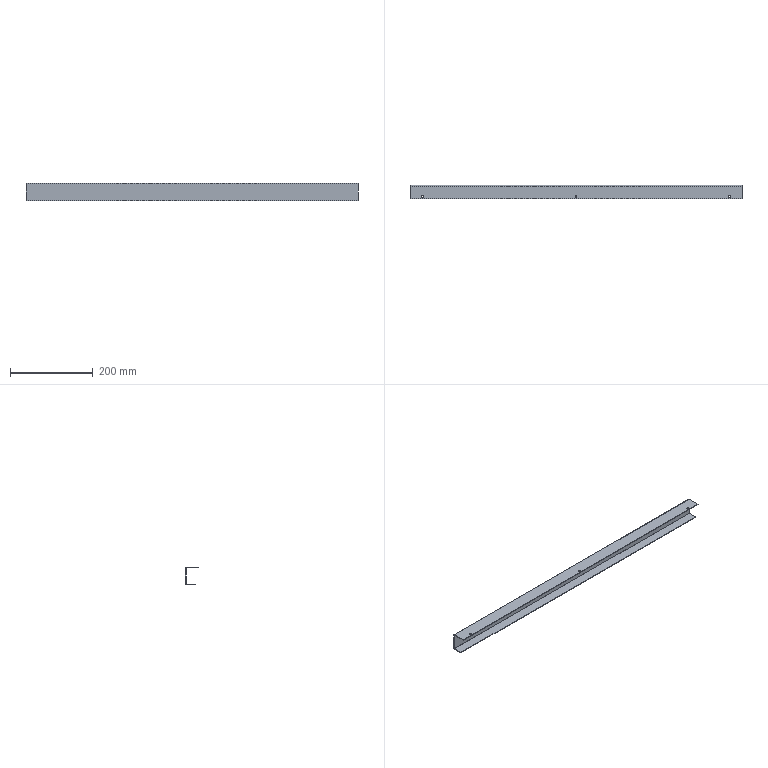Component | SolidWorks | CableChainAGuideSlot-0510-2 | 1 solid | 28 faces | box 800 x 31.5 x 43 mm | volume 113053 mm3 | plane 18 | cylinder 10 | commonest cylinder face diameters 4.5 x6 3.2 x2 0.2 x2 | material Cold Rolled Steel Sheet 08F
STEP:
#1=COLOUR_RGB('',0.7922,0.8196,0.9333);
#2=FILL_AREA_STYLE_COLOUR('',#1);
#3=FILL_AREA_STYLE('',(#2));
#4=SURFACE_STYLE_FILL_AREA(#3);
#5=SURFACE_SIDE_STYLE('',(#4));
#6=SURFACE_STYLE_USAGE(.BOTH.,#5);
#7=PRESENTATION_STYLE_ASSIGNMENT((#6));
#8=CARTESIAN_POINT('',(-31.307,2.604,135.531));
#9=VERTEX_POINT('',#8);
#10=CARTESIAN_POINT('',(-31.307,2.427,135.531));
#11=VERTEX_POINT('',#10);
#12=CARTESIAN_POINT('',(-31.307,2.515,135.531));
#13=DIRECTION('',(0.,0.,-1.));
#14=DIRECTION('',(0.,-1.,0.));
#15=AXIS2_PLACEMENT_3D('',#12,#13,#14);
#16=CIRCLE('',#15,0.08858);
#17=EDGE_CURVE('',#9,#11,#16,.T.);
#18=ORIENTED_EDGE('',*,*,#17,.F.);
#19=CARTESIAN_POINT('',(-31.307,2.604,135.472));
#20=VERTEX_POINT('',#19);
#21=CARTESIAN_POINT('',(-31.307,2.604,135.472));
#22=DIRECTION('',(0.,0.,-1.));
#23=VECTOR('',#22,39.37);
#24=LINE('',#21,#23);
#25=EDGE_CURVE('',#9,#20,#24,.T.);
#26=ORIENTED_EDGE('',*,*,#25,.T.);
#27=CARTESIAN_POINT('',(-31.307,2.427,135.472));
#28=VERTEX_POINT('',#27);
#29=CARTESIAN_POINT('',(-31.307,2.515,135.472));
#30=DIRECTION('',(0.,0.,-1.));
#31=DIRECTION('',(0.,-1.,0.));
#32=AXIS2_PLACEMENT_3D('',#29,#30,#31);
#33=CIRCLE('',#32,0.08858);
#34=EDGE_CURVE('',#20,#28,#33,.T.);
#35=ORIENTED_EDGE('',*,*,#34,.T.);
#36=CARTESIAN_POINT('',(-31.307,2.427,135.472));
#37=DIRECTION('',(0.,0.,-1.));
#38=VECTOR('',#37,39.37);
#39=LINE('',#36,#38);
#40=EDGE_CURVE('',#11,#28,#39,.T.);
#41=ORIENTED_EDGE('',*,*,#40,.F.);
#42=EDGE_LOOP('',(#18,#26,#35,#41));
#43=FACE_OUTER_BOUND('',#42,.T.);
#44=CARTESIAN_POINT('',(-31.307,2.515,135.472));
#45=DIRECTION('',(0.,0.,-1.));
#46=DIRECTION('',(0.,-1.,0.));
#47=AXIS2_PLACEMENT_3D('',#44,#45,#46);
#48=CYLINDRICAL_SURFACE('',#47,0.08858);
#49=ADVANCED_FACE('',(#43),#48,.F.);
#50=CARTESIAN_POINT('',(-60.441,2.604,135.531));
#51=VERTEX_POINT('',#50);
#52=CARTESIAN_POINT('',(-60.441,2.427,135.531));
#53=VERTEX_POINT('',#52);
#54=CARTESIAN_POINT('',(-60.441,2.515,135.531));
#55=DIRECTION('',(0.,0.,-1.));
#56=DIRECTION('',(0.,-1.,0.));
#57=AXIS2_PLACEMENT_3D('',#54,#55,#56);
#58=CIRCLE('',#57,0.08858);
#59=EDGE_CURVE('',#51,#53,#58,.T.);
#60=ORIENTED_EDGE('',*,*,#59,.F.);
#61=CARTESIAN_POINT('',(-60.441,2.604,135.472));
#62=VERTEX_POINT('',#61);
#63=CARTESIAN_POINT('',(-60.441,2.604,135.472));
#64=DIRECTION('',(0.,0.,-1.));
#65=VECTOR('',#64,39.37);
#66=LINE('',#63,#65);
#67=EDGE_CURVE('',#51,#62,#66,.T.);
#68=ORIENTED_EDGE('',*,*,#67,.T.);
#69=CARTESIAN_POINT('',(-60.441,2.427,135.472));
#70=VERTEX_POINT('',#69);
#71=CARTESIAN_POINT('',(-60.441,2.515,135.472));
#72=DIRECTION('',(0.,0.,-1.));
#73=DIRECTION('',(0.,-1.,0.));
#74=AXIS2_PLACEMENT_3D('',#71,#72,#73);
#75=CIRCLE('',#74,0.08858);
#76=EDGE_CURVE('',#62,#70,#75,.T.);
#77=ORIENTED_EDGE('',*,*,#76,.T.);
#78=CARTESIAN_POINT('',(-60.441,2.427,135.472));
#79=DIRECTION('',(0.,0.,-1.));
#80=VECTOR('',#79,39.37);
#81=LINE('',#78,#80);
#82=EDGE_CURVE('',#53,#70,#81,.T.);
#83=ORIENTED_EDGE('',*,*,#82,.F.);
#84=EDGE_LOOP('',(#60,#68,#77,#83));
#85=FACE_OUTER_BOUND('',#84,.T.);
#86=CARTESIAN_POINT('',(-60.441,2.515,135.472));
#87=DIRECTION('',(0.,0.,-1.));
#88=DIRECTION('',(0.,-1.,0.));
#89=AXIS2_PLACEMENT_3D('',#86,#87,#88);
#90=CYLINDRICAL_SURFACE('',#89,0.08858);
#91=ADVANCED_FACE('',(#85),#90,.F.);
#92=CARTESIAN_POINT('',(-45.874,2.604,135.531));
#93=VERTEX_POINT('',#92);
#94=CARTESIAN_POINT('',(-45.874,2.427,135.531));
#95=VERTEX_POINT('',#94);
#96=CARTESIAN_POINT('',(-45.874,2.515,135.531));
#97=DIRECTION('',(0.,0.,-1.));
#98=DIRECTION('',(0.,-1.,0.));
#99=AXIS2_PLACEMENT_3D('',#96,#97,#98);
#100=CIRCLE('',#99,0.08858);
#101=EDGE_CURVE('',#93,#95,#100,.T.);
#102=ORIENTED_EDGE('',*,*,#101,.F.);
#103=CARTESIAN_POINT('',(-45.874,2.604,135.472));
#104=VERTEX_POINT('',#103);
#105=CARTESIAN_POINT('',(-45.874,2.604,135.472));
#106=DIRECTION('',(0.,0.,-1.));
#107=VECTOR('',#106,39.37);
#108=LINE('',#105,#107);
#109=EDGE_CURVE('',#93,#104,#108,.T.);
#110=ORIENTED_EDGE('',*,*,#109,.T.);
#111=CARTESIAN_POINT('',(-45.874,2.427,135.472));
#112=VERTEX_POINT('',#111);
#113=CARTESIAN_POINT('',(-45.874,2.515,135.472));
#114=DIRECTION('',(0.,0.,-1.));
#115=DIRECTION('',(0.,-1.,0.));
#116=AXIS2_PLACEMENT_3D('',#113,#114,#115);
#117=CIRCLE('',#116,0.08858);
#118=EDGE_CURVE('',#104,#112,#117,.T.);
#119=ORIENTED_EDGE('',*,*,#118,.T.);
#120=CARTESIAN_POINT('',(-45.874,2.427,135.472));
#121=DIRECTION('',(0.,0.,-1.));
#122=VECTOR('',#121,39.37);
#123=LINE('',#120,#122);
#124=EDGE_CURVE('',#95,#112,#123,.T.);
#125=ORIENTED_EDGE('',*,*,#124,.F.);
#126=EDGE_LOOP('',(#102,#110,#119,#125));
#127=FACE_OUTER_BOUND('',#126,.T.);
#128=CARTESIAN_POINT('',(-45.874,2.515,135.472));
#129=DIRECTION('',(0.,0.,-1.));
#130=DIRECTION('',(0.,-1.,0.));
#131=AXIS2_PLACEMENT_3D('',#128,#129,#130);
#132=CYLINDRICAL_SURFACE('',#131,0.08858);
#133=ADVANCED_FACE('',(#127),#132,.F.);
#134=CARTESIAN_POINT('',(-61.622,3.496,133.898));
#135=VERTEX_POINT('',#134);
#136=CARTESIAN_POINT('',(-61.622,3.496,133.839));
#137=VERTEX_POINT('',#136);
#138=CARTESIAN_POINT('',(-61.622,3.496,133.898));
#139=DIRECTION('',(0.,0.,-1.));
#140=VECTOR('',#139,39.37);
#141=LINE('',#138,#140);
#142=EDGE_CURVE('',#135,#137,#141,.T.);
#143=ORIENTED_EDGE('',*,*,#142,.F.);
#144=CARTESIAN_POINT('',(-61.622,3.5,133.902));
#145=VERTEX_POINT('',#144);
#146=CARTESIAN_POINT('',(-61.622,3.496,133.902));
#147=DIRECTION('',(1.,0.,0.));
#148=DIRECTION('',(0.,1.,0.));
#149=AXIS2_PLACEMENT_3D('',#146,#147,#148);
#150=CIRCLE('',#149,0.003937);
#151=EDGE_CURVE('',#135,#145,#150,.T.);
#152=ORIENTED_EDGE('',*,*,#151,.T.);
#153=CARTESIAN_POINT('',(-61.622,3.559,133.902));
#154=VERTEX_POINT('',#153);
#155=CARTESIAN_POINT('',(-61.622,3.559,133.902));
#156=DIRECTION('',(0.,-1.,0.));
#157=VECTOR('',#156,39.37);
#158=LINE('',#155,#157);
#159=EDGE_CURVE('',#154,#145,#158,.T.);
#160=ORIENTED_EDGE('',*,*,#159,.F.);
#161=CARTESIAN_POINT('',(-61.622,3.496,133.902));
#162=DIRECTION('',(1.,0.,0.));
#163=DIRECTION('',(0.,0.,-1.));
#164=AXIS2_PLACEMENT_3D('',#161,#162,#163);
#165=CIRCLE('',#164,0.06299);
#166=EDGE_CURVE('',#137,#154,#165,.T.);
#167=ORIENTED_EDGE('',*,*,#166,.F.);
#168=EDGE_LOOP('',(#143,#152,#160,#167));
#169=FACE_OUTER_BOUND('',#168,.T.);
#170=CARTESIAN_POINT('',(-61.622,3.496,133.898));
#171=DIRECTION('',(-1.,0.,0.));
#172=DIRECTION('',(0.,1.,0.));
#173=AXIS2_PLACEMENT_3D('',#170,#171,#172);
#174=PLANE('',#173);
#175=ADVANCED_FACE('',(#169),#174,.T.);
#176=CARTESIAN_POINT('',(-61.622,2.634,133.898));
#177=VERTEX_POINT('',#176);
#178=CARTESIAN_POINT('',(-61.622,3.5,133.898));
#179=DIRECTION('',(0.,1.,0.));
#180=VECTOR('',#179,39.37);
#181=LINE('',#178,#180);
#182=EDGE_CURVE('',#177,#135,#181,.T.);
#183=ORIENTED_EDGE('',*,*,#182,.T.);
#184=ORIENTED_EDGE('',*,*,#142,.T.);
#185=CARTESIAN_POINT('',(-61.622,2.634,133.839));
#186=VERTEX_POINT('',#185);
#187=CARTESIAN_POINT('',(-61.622,3.5,133.839));
#188=DIRECTION('',(0.,1.,0.));
#189=VECTOR('',#188,39.37);
#190=LINE('',#187,#189);
#191=EDGE_CURVE('',#186,#137,#190,.T.);
#192=ORIENTED_EDGE('',*,*,#191,.F.);
#193=CARTESIAN_POINT('',(-61.622,2.634,133.898));
#194=DIRECTION('',(0.,0.,-1.));
#195=VECTOR('',#194,39.37);
#196=LINE('',#193,#195);
#197=EDGE_CURVE('',#177,#186,#196,.T.);
#198=ORIENTED_EDGE('',*,*,#197,.F.);
#199=EDGE_LOOP('',(#183,#184,#192,#198));
#200=FACE_OUTER_BOUND('',#199,.T.);
#201=CARTESIAN_POINT('',(-61.622,3.559,133.902));
#202=DIRECTION('',(-1.,0.,0.));
#203=DIRECTION('',(0.,1.,0.));
#204=AXIS2_PLACEMENT_3D('',#201,#202,#203);
#205=PLANE('',#204);
#206=ADVANCED_FACE('',(#200),#205,.T.);
#207=CARTESIAN_POINT('',(-30.126,3.5,133.902));
#208=VERTEX_POINT('',#207);
#209=CARTESIAN_POINT('',(-30.126,3.559,133.902));
#210=VERTEX_POINT('',#209);
#211=CARTESIAN_POINT('',(-30.126,3.5,133.902));
#212=DIRECTION('',(0.,1.,0.));
#213=VECTOR('',#212,39.37);
#214=LINE('',#211,#213);
#215=EDGE_CURVE('',#208,#210,#214,.T.);
#216=ORIENTED_EDGE('',*,*,#215,.F.);
#217=CARTESIAN_POINT('',(-30.126,3.496,133.898));
#218=VERTEX_POINT('',#217);
#219=CARTESIAN_POINT('',(-30.126,3.496,133.902));
#220=DIRECTION('',(1.,0.,0.));
#221=DIRECTION('',(0.,1.,0.));
#222=AXIS2_PLACEMENT_3D('',#219,#220,#221);
#223=CIRCLE('',#222,0.003937);
#224=EDGE_CURVE('',#218,#208,#223,.T.);
#225=ORIENTED_EDGE('',*,*,#224,.F.);
#226=CARTESIAN_POINT('',(-30.126,3.496,133.839));
#227=VERTEX_POINT('',#226);
#228=CARTESIAN_POINT('',(-30.126,3.496,133.839));
#229=DIRECTION('',(0.,0.,1.));
#230=VECTOR('',#229,39.37);
#231=LINE('',#228,#230);
#232=EDGE_CURVE('',#227,#218,#231,.T.);
#233=ORIENTED_EDGE('',*,*,#232,.F.);
#234=CARTESIAN_POINT('',(-30.126,3.496,133.902));
#235=DIRECTION('',(1.,0.,0.));
#236=DIRECTION('',(0.,0.,-1.));
#237=AXIS2_PLACEMENT_3D('',#234,#235,#236);
#238=CIRCLE('',#237,0.06299);
#239=EDGE_CURVE('',#227,#210,#238,.T.);
#240=ORIENTED_EDGE('',*,*,#239,.T.);
#241=EDGE_LOOP('',(#216,#225,#233,#240));
#242=FACE_OUTER_BOUND('',#241,.T.);
#243=CARTESIAN_POINT('',(-30.126,3.5,133.902));
#244=DIRECTION('',(1.,0.,0.));
#245=DIRECTION('',(0.,-1.,0.));
#246=AXIS2_PLACEMENT_3D('',#243,#244,#245);
#247=PLANE('',#246);
#248=ADVANCED_FACE('',(#242),#247,.T.);
#249=CARTESIAN_POINT('',(-30.126,3.5,135.469));
#250=VERTEX_POINT('',#249);
#251=CARTESIAN_POINT('',(-30.126,3.5,135.472));
#252=DIRECTION('',(0.,0.,1.));
#253=VECTOR('',#252,39.37);
#254=LINE('',#251,#253);
#255=EDGE_CURVE('',#208,#250,#254,.T.);
#256=ORIENTED_EDGE('',*,*,#255,.F.);
#257=ORIENTED_EDGE('',*,*,#215,.T.);
#258=CARTESIAN_POINT('',(-30.126,3.559,135.469));
#259=VERTEX_POINT('',#258);
#260=CARTESIAN_POINT('',(-30.126,3.559,135.472));
#261=DIRECTION('',(0.,0.,1.));
#262=VECTOR('',#261,39.37);
#263=LINE('',#260,#262);
#264=EDGE_CURVE('',#210,#259,#263,.T.);
#265=ORIENTED_EDGE('',*,*,#264,.T.);
#266=CARTESIAN_POINT('',(-30.126,3.559,135.469));
#267=DIRECTION('',(0.,-1.,0.));
#268=VECTOR('',#267,39.37);
#269=LINE('',#266,#268);
#270=EDGE_CURVE('',#259,#250,#269,.T.);
#271=ORIENTED_EDGE('',*,*,#270,.T.);
#272=EDGE_LOOP('',(#256,#257,#265,#271));
#273=FACE_OUTER_BOUND('',#272,.T.);
#274=CARTESIAN_POINT('',(-30.126,3.496,133.839));
#275=DIRECTION('',(1.,0.,0.));
#276=DIRECTION('',(0.,-1.,0.));
#277=AXIS2_PLACEMENT_3D('',#274,#275,#276);
#278=PLANE('',#277);
#279=ADVANCED_FACE('',(#273),#278,.T.);
#280=CARTESIAN_POINT('',(-61.622,3.5,135.469));
#281=VERTEX_POINT('',#280);
#282=CARTESIAN_POINT('',(-61.622,3.559,135.469));
#283=VERTEX_POINT('',#282);
#284=CARTESIAN_POINT('',(-61.622,3.5,135.469));
#285=DIRECTION('',(0.,1.,0.));
#286=VECTOR('',#285,39.37);
#287=LINE('',#284,#286);
#288=EDGE_CURVE('',#281,#283,#287,.T.);
#289=ORIENTED_EDGE('',*,*,#288,.F.);
#290=CARTESIAN_POINT('',(-61.622,3.496,135.472));
#291=VERTEX_POINT('',#290);
#292=CARTESIAN_POINT('',(-61.622,3.496,135.469));
#293=DIRECTION('',(1.,0.,0.));
#294=DIRECTION('',(0.,1.,0.));
#295=AXIS2_PLACEMENT_3D('',#292,#293,#294);
#296=CIRCLE('',#295,0.003937);
#297=EDGE_CURVE('',#281,#291,#296,.T.);
#298=ORIENTED_EDGE('',*,*,#297,.T.);
#299=CARTESIAN_POINT('',(-61.622,3.496,135.531));
#300=VERTEX_POINT('',#299);
#301=CARTESIAN_POINT('',(-61.622,3.496,135.531));
#302=DIRECTION('',(0.,0.,-1.));
#303=VECTOR('',#302,39.37);
#304=LINE('',#301,#303);
#305=EDGE_CURVE('',#300,#291,#304,.T.);
#306=ORIENTED_EDGE('',*,*,#305,.F.);
#307=CARTESIAN_POINT('',(-61.622,3.496,135.469));
#308=DIRECTION('',(1.,0.,0.));
#309=DIRECTION('',(0.,0.,-1.));
#310=AXIS2_PLACEMENT_3D('',#307,#308,#309);
#311=CIRCLE('',#310,0.06299);
#312=EDGE_CURVE('',#283,#300,#311,.T.);
#313=ORIENTED_EDGE('',*,*,#312,.F.);
#314=EDGE_LOOP('',(#289,#298,#306,#313));
#315=FACE_OUTER_BOUND('',#314,.T.);
#316=CARTESIAN_POINT('',(-61.622,3.5,135.469));
#317=DIRECTION('',(-1.,0.,0.));
#318=DIRECTION('',(0.,1.,0.));
#319=AXIS2_PLACEMENT_3D('',#316,#317,#318);
#320=PLANE('',#319);
#321=ADVANCED_FACE('',(#315),#320,.T.);
#322=CARTESIAN_POINT('',(-61.622,3.5,135.472));
#323=DIRECTION('',(0.,0.,1.));
#324=VECTOR('',#323,39.37);
#325=LINE('',#322,#324);
#326=EDGE_CURVE('',#145,#281,#325,.T.);
#327=ORIENTED_EDGE('',*,*,#326,.T.);
#328=ORIENTED_EDGE('',*,*,#288,.T.);
#329=CARTESIAN_POINT('',(-61.622,3.559,135.472));
#330=DIRECTION('',(0.,0.,1.));
#331=VECTOR('',#330,39.37);
#332=LINE('',#329,#331);
#333=EDGE_CURVE('',#154,#283,#332,.T.);
#334=ORIENTED_EDGE('',*,*,#333,.F.);
#335=ORIENTED_EDGE('',*,*,#159,.T.);
#336=EDGE_LOOP('',(#327,#328,#334,#335));
#337=FACE_OUTER_BOUND('',#336,.T.);
#338=CARTESIAN_POINT('',(-61.622,3.496,135.531));
#339=DIRECTION('',(-1.,0.,0.));
#340=DIRECTION('',(0.,1.,0.));
#341=AXIS2_PLACEMENT_3D('',#338,#339,#340);
#342=PLANE('',#341);
#343=ADVANCED_FACE('',(#337),#342,.T.);
#344=CARTESIAN_POINT('',(-30.126,3.496,135.472));
#345=VERTEX_POINT('',#344);
#346=CARTESIAN_POINT('',(-30.126,3.496,135.531));
#347=VERTEX_POINT('',#346);
#348=CARTESIAN_POINT('',(-30.126,3.496,135.472));
#349=DIRECTION('',(0.,0.,1.));
#350=VECTOR('',#349,39.37);
#351=LINE('',#348,#350);
#352=EDGE_CURVE('',#345,#347,#351,.T.);
#353=ORIENTED_EDGE('',*,*,#352,.F.);
#354=CARTESIAN_POINT('',(-30.126,3.496,135.469));
#355=DIRECTION('',(1.,0.,0.));
#356=DIRECTION('',(0.,1.,0.));
#357=AXIS2_PLACEMENT_3D('',#354,#355,#356);
#358=CIRCLE('',#357,0.003937);
#359=EDGE_CURVE('',#250,#345,#358,.T.);
#360=ORIENTED_EDGE('',*,*,#359,.F.);
#361=ORIENTED_EDGE('',*,*,#270,.F.);
#362=CARTESIAN_POINT('',(-30.126,3.496,135.469));
#363=DIRECTION('',(1.,0.,0.));
#364=DIRECTION('',(0.,0.,-1.));
#365=AXIS2_PLACEMENT_3D('',#362,#363,#364);
#366=CIRCLE('',#365,0.06299);
#367=EDGE_CURVE('',#259,#347,#366,.T.);
#368=ORIENTED_EDGE('',*,*,#367,.T.);
#369=EDGE_LOOP('',(#353,#360,#361,#368));
#370=FACE_OUTER_BOUND('',#369,.T.);
#371=CARTESIAN_POINT('',(-30.126,3.496,135.472));
#372=DIRECTION('',(1.,0.,0.));
#373=DIRECTION('',(0.,-1.,0.));
#374=AXIS2_PLACEMENT_3D('',#371,#372,#373);
#375=PLANE('',#374);
#376=ADVANCED_FACE('',(#370),#375,.T.);
#377=CARTESIAN_POINT('',(-30.126,2.319,135.472));
#378=VERTEX_POINT('',#377);
#379=CARTESIAN_POINT('',(-30.126,3.5,135.472));
#380=DIRECTION('',(0.,-1.,0.));
#381=VECTOR('',#380,39.37);
#382=LINE('',#379,#381);
#383=EDGE_CURVE('',#345,#378,#382,.T.);
#384=ORIENTED_EDGE('',*,*,#383,.F.);
#385=ORIENTED_EDGE('',*,*,#352,.T.);
#386=CARTESIAN_POINT('',(-30.126,2.319,135.531));
#387=VERTEX_POINT('',#386);
#388=CARTESIAN_POINT('',(-30.126,3.5,135.531));
#389=DIRECTION('',(0.,-1.,0.));
#390=VECTOR('',#389,39.37);
#391=LINE('',#388,#390);
#392=EDGE_CURVE('',#347,#387,#391,.T.);
#393=ORIENTED_EDGE('',*,*,#392,.T.);
#394=CARTESIAN_POINT('',(-30.126,2.319,135.531));
#395=DIRECTION('',(0.,0.,-1.));
#396=VECTOR('',#395,39.37);
#397=LINE('',#394,#396);
#398=EDGE_CURVE('',#387,#378,#397,.T.);
#399=ORIENTED_EDGE('',*,*,#398,.T.);
#400=EDGE_LOOP('',(#384,#385,#393,#399));
#401=FACE_OUTER_BOUND('',#400,.T.);
#402=CARTESIAN_POINT('',(-30.126,3.559,135.469));
#403=DIRECTION('',(1.,0.,0.));
#404=DIRECTION('',(0.,-1.,0.));
#405=AXIS2_PLACEMENT_3D('',#402,#403,#404);
#406=PLANE('',#405);
#407=ADVANCED_FACE('',(#401),#406,.T.);
#408=CARTESIAN_POINT('',(-31.307,2.515,135.472));
#409=DIRECTION('',(0.,0.,-1.));
#410=DIRECTION('',(0.,-1.,0.));
#411=AXIS2_PLACEMENT_3D('',#408,#409,#410);
#412=CIRCLE('',#411,0.08858);
#413=EDGE_CURVE('',#28,#20,#412,.T.);
#414=ORIENTED_EDGE('',*,*,#413,.F.);
#415=ORIENTED_EDGE('',*,*,#34,.F.);
#416=EDGE_LOOP('',(#414,#415));
#417=FACE_BOUND('',#416,.T.);
#418=CARTESIAN_POINT('',(-60.441,2.515,135.472));
#419=DIRECTION('',(0.,0.,-1.));
#420=DIRECTION('',(0.,-1.,0.));
#421=AXIS2_PLACEMENT_3D('',#418,#419,#420);
#422=CIRCLE('',#421,0.08858);
#423=EDGE_CURVE('',#70,#62,#422,.T.);
#424=ORIENTED_EDGE('',*,*,#423,.F.);
#425=ORIENTED_EDGE('',*,*,#76,.F.);
#426=EDGE_LOOP('',(#424,#425));
#427=FACE_BOUND('',#426,.T.);
#428=CARTESIAN_POINT('',(-45.874,2.515,135.472));
#429=DIRECTION('',(0.,0.,-1.));
#430=DIRECTION('',(0.,-1.,0.));
#431=AXIS2_PLACEMENT_3D('',#428,#429,#430);
#432=CIRCLE('',#431,0.08858);
#433=EDGE_CURVE('',#112,#104,#432,.T.);
#434=ORIENTED_EDGE('',*,*,#433,.F.);
#435=ORIENTED_EDGE('',*,*,#118,.F.);
#436=EDGE_LOOP('',(#434,#435));
#437=FACE_BOUND('',#436,.T.);
#438=ORIENTED_EDGE('',*,*,#383,.T.);
#439=CARTESIAN_POINT('',(-61.622,2.319,135.472));
#440=VERTEX_POINT('',#439);
#441=CARTESIAN_POINT('',(-61.622,2.319,135.472));
#442=DIRECTION('',(1.,0.,0.));
#443=VECTOR('',#442,39.37);
#444=LINE('',#441,#443);
#445=EDGE_CURVE('',#440,#378,#444,.T.);
#446=ORIENTED_EDGE('',*,*,#445,.F.);
#447=CARTESIAN_POINT('',(-61.622,3.5,135.472));
#448=DIRECTION('',(0.,-1.,0.));
#449=VECTOR('',#448,39.37);
#450=LINE('',#447,#449);
#451=EDGE_CURVE('',#291,#440,#450,.T.);
#452=ORIENTED_EDGE('',*,*,#451,.F.);
#453=CARTESIAN_POINT('',(-61.622,3.496,135.472));
#454=DIRECTION('',(1.,0.,0.));
#455=VECTOR('',#454,39.37);
#456=LINE('',#453,#455);
#457=EDGE_CURVE('',#291,#345,#456,.T.);
#458=ORIENTED_EDGE('',*,*,#457,.T.);
#459=EDGE_LOOP('',(#438,#446,#452,#458));
#460=FACE_OUTER_BOUND('',#459,.T.);
#461=CARTESIAN_POINT('',(-61.622,3.5,135.472));
#462=DIRECTION('',(0.,0.,1.));
#463=DIRECTION('',(0.,1.,0.));
#464=AXIS2_PLACEMENT_3D('',#461,#462,#463);
#465=PLANE('',#464);
#466=ADVANCED_FACE('',(#417,#427,#437,#460),#465,.F.);
#467=ORIENTED_EDGE('',*,*,#398,.F.);
#468=CARTESIAN_POINT('',(-61.622,2.319,135.531));
#469=VERTEX_POINT('',#468);
#470=CARTESIAN_POINT('',(-61.622,2.319,135.531));
#471=DIRECTION('',(1.,0.,0.));
#472=VECTOR('',#471,39.37);
#473=LINE('',#470,#472);
#474=EDGE_CURVE('',#469,#387,#473,.T.);
#475=ORIENTED_EDGE('',*,*,#474,.F.);
#476=CARTESIAN_POINT('',(-61.622,2.319,135.531));
#477=DIRECTION('',(0.,0.,-1.));
#478=VECTOR('',#477,39.37);
#479=LINE('',#476,#478);
#480=EDGE_CURVE('',#469,#440,#479,.T.);
#481=ORIENTED_EDGE('',*,*,#480,.T.);
#482=ORIENTED_EDGE('',*,*,#445,.T.);
#483=EDGE_LOOP('',(#467,#475,#481,#482));
#484=FACE_OUTER_BOUND('',#483,.T.);
#485=CARTESIAN_POINT('',(-61.622,2.319,135.531));
#486=DIRECTION('',(0.,-1.,0.));
#487=DIRECTION('',(0.,0.,1.));
#488=AXIS2_PLACEMENT_3D('',#485,#486,#487);
#489=PLANE('',#488);
#490=ADVANCED_FACE('',(#484),#489,.T.);
#491=CARTESIAN_POINT('',(-31.307,2.515,135.531));
#492=DIRECTION('',(0.,0.,-1.));
#493=DIRECTION('',(0.,-1.,0.));
#494=AXIS2_PLACEMENT_3D('',#491,#492,#493);
#495=CIRCLE('',#494,0.08858);
#496=EDGE_CURVE('',#11,#9,#495,.T.);
#497=ORIENTED_EDGE('',*,*,#496,.T.);
#498=ORIENTED_EDGE('',*,*,#17,.T.);
#499=EDGE_LOOP('',(#497,#498));
#500=FACE_BOUND('',#499,.T.);
#501=CARTESIAN_POINT('',(-60.441,2.515,135.531));
#502=DIRECTION('',(0.,0.,-1.));
#503=DIRECTION('',(0.,-1.,0.));
#504=AXIS2_PLACEMENT_3D('',#501,#502,#503);
#505=CIRCLE('',#504,0.08858);
#506=EDGE_CURVE('',#53,#51,#505,.T.);
#507=ORIENTED_EDGE('',*,*,#506,.T.);
#508=ORIENTED_EDGE('',*,*,#59,.T.);
#509=EDGE_LOOP('',(#507,#508));
#510=FACE_BOUND('',#509,.T.);
#511=CARTESIAN_POINT('',(-45.874,2.515,135.531));
#512=DIRECTION('',(0.,0.,-1.));
#513=DIRECTION('',(0.,-1.,0.));
#514=AXIS2_PLACEMENT_3D('',#511,#512,#513);
#515=CIRCLE('',#514,0.08858);
#516=EDGE_CURVE('',#95,#93,#515,.T.);
#517=ORIENTED_EDGE('',*,*,#516,.T.);
#518=ORIENTED_EDGE('',*,*,#101,.T.);
#519=EDGE_LOOP('',(#517,#518));
#520=FACE_BOUND('',#519,.T.);
#521=ORIENTED_EDGE('',*,*,#392,.F.);
#522=CARTESIAN_POINT('',(-61.622,3.496,135.531));
#523=DIRECTION('',(1.,0.,0.));
#524=VECTOR('',#523,39.37);
#525=LINE('',#522,#524);
#526=EDGE_CURVE('',#300,#347,#525,.T.);
#527=ORIENTED_EDGE('',*,*,#526,.F.);
#528=CARTESIAN_POINT('',(-61.622,3.5,135.531));
#529=DIRECTION('',(0.,-1.,0.));
#530=VECTOR('',#529,39.37);
#531=LINE('',#528,#530);
#532=EDGE_CURVE('',#300,#469,#531,.T.);
#533=ORIENTED_EDGE('',*,*,#532,.T.);
#534=ORIENTED_EDGE('',*,*,#474,.T.);
#535=EDGE_LOOP('',(#521,#527,#533,#534));
#536=FACE_OUTER_BOUND('',#535,.T.);
#537=CARTESIAN_POINT('',(-61.622,3.5,135.531));
#538=DIRECTION('',(0.,0.,1.));
#539=DIRECTION('',(0.,1.,0.));
#540=AXIS2_PLACEMENT_3D('',#537,#538,#539);
#541=PLANE('',#540);
#542=ADVANCED_FACE('',(#500,#510,#520,#536),#541,.T.);
#543=ORIENTED_EDGE('',*,*,#367,.F.);
#544=CARTESIAN_POINT('',(-61.622,3.559,135.469));
#545=DIRECTION('',(1.,0.,0.));
#546=VECTOR('',#545,39.37);
#547=LINE('',#544,#546);
#548=EDGE_CURVE('',#283,#259,#547,.T.);
#549=ORIENTED_EDGE('',*,*,#548,.F.);
#550=ORIENTED_EDGE('',*,*,#312,.T.);
#551=ORIENTED_EDGE('',*,*,#526,.T.);
#552=EDGE_LOOP('',(#543,#549,#550,#551));
#553=FACE_OUTER_BOUND('',#552,.T.);
#554=CARTESIAN_POINT('',(-61.622,3.496,135.469));
#555=DIRECTION('',(1.,0.,0.));
#556=DIRECTION('',(0.,-1.,0.));
#557=AXIS2_PLACEMENT_3D('',#554,#555,#556);
#558=CYLINDRICAL_SURFACE('',#557,0.06299);
#559=ADVANCED_FACE('',(#553),#558,.T.);
#560=ORIENTED_EDGE('',*,*,#264,.F.);
#561=CARTESIAN_POINT('',(-61.622,3.559,133.902));
#562=DIRECTION('',(1.,0.,0.));
#563=VECTOR('',#562,39.37);
#564=LINE('',#561,#563);
#565=EDGE_CURVE('',#154,#210,#564,.T.);
#566=ORIENTED_EDGE('',*,*,#565,.F.);
#567=ORIENTED_EDGE('',*,*,#333,.T.);
#568=ORIENTED_EDGE('',*,*,#548,.T.);
#569=EDGE_LOOP('',(#560,#566,#567,#568));
#570=FACE_OUTER_BOUND('',#569,.T.);
#571=CARTESIAN_POINT('',(-61.622,3.559,135.472));
#572=DIRECTION('',(0.,1.,0.));
#573=DIRECTION('',(0.,0.,-1.));
#574=AXIS2_PLACEMENT_3D('',#571,#572,#573);
#575=PLANE('',#574);
#576=ADVANCED_FACE('',(#570),#575,.T.);
#577=ORIENTED_EDGE('',*,*,#239,.F.);
#578=CARTESIAN_POINT('',(-61.622,3.496,133.839));
#579=DIRECTION('',(1.,0.,0.));
#580=VECTOR('',#579,39.37);
#581=LINE('',#578,#580);
#582=EDGE_CURVE('',#137,#227,#581,.T.);
#583=ORIENTED_EDGE('',*,*,#582,.F.);
#584=ORIENTED_EDGE('',*,*,#166,.T.);
#585=ORIENTED_EDGE('',*,*,#565,.T.);
#586=EDGE_LOOP('',(#577,#583,#584,#585));
#587=FACE_OUTER_BOUND('',#586,.T.);
#588=CARTESIAN_POINT('',(-61.622,3.496,133.902));
#589=DIRECTION('',(1.,0.,0.));
#590=DIRECTION('',(0.,-1.,0.));
#591=AXIS2_PLACEMENT_3D('',#588,#589,#590);
#592=CYLINDRICAL_SURFACE('',#591,0.06299);
#593=ADVANCED_FACE('',(#587),#592,.T.);
#594=CARTESIAN_POINT('',(-30.126,2.634,133.839));
#595=VERTEX_POINT('',#594);
#596=CARTESIAN_POINT('',(-30.126,3.5,133.839));
#597=DIRECTION('',(0.,1.,0.));
#598=VECTOR('',#597,39.37);
#599=LINE('',#596,#598);
#600=EDGE_CURVE('',#595,#227,#599,.T.);
#601=ORIENTED_EDGE('',*,*,#600,.F.);
#602=CARTESIAN_POINT('',(-61.622,2.634,133.839));
#603=DIRECTION('',(1.,0.,0.));
#604=VECTOR('',#603,39.37);
#605=LINE('',#602,#604);
#606=EDGE_CURVE('',#186,#595,#605,.T.);
#607=ORIENTED_EDGE('',*,*,#606,.F.);
#608=ORIENTED_EDGE('',*,*,#191,.T.);
#609=ORIENTED_EDGE('',*,*,#582,.T.);
#610=EDGE_LOOP('',(#601,#607,#608,#609));
#611=FACE_OUTER_BOUND('',#610,.T.);
#612=CARTESIAN_POINT('',(-61.622,3.5,133.839));
#613=DIRECTION('',(0.,0.,-1.));
#614=DIRECTION('',(0.,-1.,0.));
#615=AXIS2_PLACEMENT_3D('',#612,#613,#614);
#616=PLANE('',#615);
#617=ADVANCED_FACE('',(#611),#616,.T.);
#618=CARTESIAN_POINT('',(-30.126,2.634,133.898));
#619=VERTEX_POINT('',#618);
#620=CARTESIAN_POINT('',(-30.126,2.634,133.898));
#621=DIRECTION('',(0.,0.,-1.));
#622=VECTOR('',#621,39.37);
#623=LINE('',#620,#622);
#624=EDGE_CURVE('',#619,#595,#623,.T.);
#625=ORIENTED_EDGE('',*,*,#624,.F.);
#626=CARTESIAN_POINT('',(-61.622,2.634,133.898));
#627=DIRECTION('',(1.,0.,0.));
#628=VECTOR('',#627,39.37);
#629=LINE('',#626,#628);
#630=EDGE_CURVE('',#177,#619,#629,.T.);
#631=ORIENTED_EDGE('',*,*,#630,.F.);
#632=ORIENTED_EDGE('',*,*,#197,.T.);
#633=ORIENTED_EDGE('',*,*,#606,.T.);
#634=EDGE_LOOP('',(#625,#631,#632,#633));
#635=FACE_OUTER_BOUND('',#634,.T.);
#636=CARTESIAN_POINT('',(-61.622,2.634,133.898));
#637=DIRECTION('',(0.,-1.,0.));
#638=DIRECTION('',(0.,0.,1.));
#639=AXIS2_PLACEMENT_3D('',#636,#637,#638);
#640=PLANE('',#639);
#641=ADVANCED_FACE('',(#635),#640,.T.);
#642=CARTESIAN_POINT('',(-30.126,3.5,133.898));
#643=DIRECTION('',(0.,1.,0.));
#644=VECTOR('',#643,39.37);
#645=LINE('',#642,#644);
#646=EDGE_CURVE('',#619,#218,#645,.T.);
#647=ORIENTED_EDGE('',*,*,#646,.T.);
#648=CARTESIAN_POINT('',(-61.622,3.496,133.898));
#649=DIRECTION('',(1.,0.,0.));
#650=VECTOR('',#649,39.37);
#651=LINE('',#648,#650);
#652=EDGE_CURVE('',#135,#218,#651,.T.);
#653=ORIENTED_EDGE('',*,*,#652,.F.);
#654=ORIENTED_EDGE('',*,*,#182,.F.);
#655=ORIENTED_EDGE('',*,*,#630,.T.);
#656=EDGE_LOOP('',(#647,#653,#654,#655));
#657=FACE_OUTER_BOUND('',#656,.T.);
#658=CARTESIAN_POINT('',(-61.622,3.5,133.898));
#659=DIRECTION('',(0.,0.,-1.));
#660=DIRECTION('',(0.,-1.,0.));
#661=AXIS2_PLACEMENT_3D('',#658,#659,#660);
#662=PLANE('',#661);
#663=ADVANCED_FACE('',(#657),#662,.F.);
#664=ORIENTED_EDGE('',*,*,#224,.T.);
#665=CARTESIAN_POINT('',(-61.622,3.5,133.902));
#666=DIRECTION('',(1.,0.,0.));
#667=VECTOR('',#666,39.37);
#668=LINE('',#665,#667);
#669=EDGE_CURVE('',#145,#208,#668,.T.);
#670=ORIENTED_EDGE('',*,*,#669,.F.);
#671=ORIENTED_EDGE('',*,*,#151,.F.);
#672=ORIENTED_EDGE('',*,*,#652,.T.);
#673=EDGE_LOOP('',(#664,#670,#671,#672));
#674=FACE_OUTER_BOUND('',#673,.T.);
#675=CARTESIAN_POINT('',(-61.622,3.496,133.902));
#676=DIRECTION('',(1.,0.,0.));
#677=DIRECTION('',(0.,-1.,0.));
#678=AXIS2_PLACEMENT_3D('',#675,#676,#677);
#679=CYLINDRICAL_SURFACE('',#678,0.003937);
#680=ADVANCED_FACE('',(#674),#679,.F.);
#681=ORIENTED_EDGE('',*,*,#255,.T.);
#682=CARTESIAN_POINT('',(-61.622,3.5,135.469));
#683=DIRECTION('',(1.,0.,0.));
#684=VECTOR('',#683,39.37);
#685=LINE('',#682,#684);
#686=EDGE_CURVE('',#281,#250,#685,.T.);
#687=ORIENTED_EDGE('',*,*,#686,.F.);
#688=ORIENTED_EDGE('',*,*,#326,.F.);
#689=ORIENTED_EDGE('',*,*,#669,.T.);
#690=EDGE_LOOP('',(#681,#687,#688,#689));
#691=FACE_OUTER_BOUND('',#690,.T.);
#692=CARTESIAN_POINT('',(-61.622,3.5,135.472));
#693=DIRECTION('',(0.,1.,0.));
#694=DIRECTION('',(0.,0.,-1.));
#695=AXIS2_PLACEMENT_3D('',#692,#693,#694);
#696=PLANE('',#695);
#697=ADVANCED_FACE('',(#691),#696,.F.);
#698=ORIENTED_EDGE('',*,*,#359,.T.);
#699=ORIENTED_EDGE('',*,*,#457,.F.);
#700=ORIENTED_EDGE('',*,*,#297,.F.);
#701=ORIENTED_EDGE('',*,*,#686,.T.);
#702=EDGE_LOOP('',(#698,#699,#700,#701));
#703=FACE_OUTER_BOUND('',#702,.T.);
#704=CARTESIAN_POINT('',(-61.622,3.496,135.469));
#705=DIRECTION('',(1.,0.,0.));
#706=DIRECTION('',(0.,-1.,0.));
#707=AXIS2_PLACEMENT_3D('',#704,#705,#706);
#708=CYLINDRICAL_SURFACE('',#707,0.003937);
#709=ADVANCED_FACE('',(#703),#708,.F.);
#710=ORIENTED_EDGE('',*,*,#451,.T.);
#711=ORIENTED_EDGE('',*,*,#480,.F.);
#712=ORIENTED_EDGE('',*,*,#532,.F.);
#713=ORIENTED_EDGE('',*,*,#305,.T.);
#714=EDGE_LOOP('',(#710,#711,#712,#713));
#715=FACE_OUTER_BOUND('',#714,.T.);
#716=CARTESIAN_POINT('',(-61.622,3.496,135.469));
#717=DIRECTION('',(-1.,0.,0.));
#718=DIRECTION('',(0.,0.,-1.));
#719=AXIS2_PLACEMENT_3D('',#716,#717,#718);
#720=PLANE('',#719);
#721=ADVANCED_FACE('',(#715),#720,.T.);
#722=ORIENTED_EDGE('',*,*,#600,.T.);
#723=ORIENTED_EDGE('',*,*,#232,.T.);
#724=ORIENTED_EDGE('',*,*,#646,.F.);
#725=ORIENTED_EDGE('',*,*,#624,.T.);
#726=EDGE_LOOP('',(#722,#723,#724,#725));
#727=FACE_OUTER_BOUND('',#726,.T.);
#728=CARTESIAN_POINT('',(-30.126,3.496,135.469));
#729=DIRECTION('',(-1.,0.,0.));
#730=DIRECTION('',(0.,0.,-1.));
#731=AXIS2_PLACEMENT_3D('',#728,#729,#730);
#732=PLANE('',#731);
#733=ADVANCED_FACE('',(#727),#732,.F.);
#734=ORIENTED_EDGE('',*,*,#109,.F.);
#735=ORIENTED_EDGE('',*,*,#516,.F.);
#736=ORIENTED_EDGE('',*,*,#124,.T.);
#737=ORIENTED_EDGE('',*,*,#433,.T.);
#738=EDGE_LOOP('',(#734,#735,#736,#737));
#739=FACE_OUTER_BOUND('',#738,.T.);
#740=CARTESIAN_POINT('',(-45.874,2.515,135.472));
#741=DIRECTION('',(0.,0.,-1.));
#742=DIRECTION('',(0.,-1.,0.));
#743=AXIS2_PLACEMENT_3D('',#740,#741,#742);
#744=CYLINDRICAL_SURFACE('',#743,0.08858);
#745=ADVANCED_FACE('',(#739),#744,.F.);
#746=ORIENTED_EDGE('',*,*,#67,.F.);
#747=ORIENTED_EDGE('',*,*,#506,.F.);
#748=ORIENTED_EDGE('',*,*,#82,.T.);
#749=ORIENTED_EDGE('',*,*,#423,.T.);
#750=EDGE_LOOP('',(#746,#747,#748,#749));
#751=FACE_OUTER_BOUND('',#750,.T.);
#752=CARTESIAN_POINT('',(-60.441,2.515,135.472));
#753=DIRECTION('',(0.,0.,-1.));
#754=DIRECTION('',(0.,-1.,0.));
#755=AXIS2_PLACEMENT_3D('',#752,#753,#754);
#756=CYLINDRICAL_SURFACE('',#755,0.08858);
#757=ADVANCED_FACE('',(#751),#756,.F.);
#758=ORIENTED_EDGE('',*,*,#25,.F.);
#759=ORIENTED_EDGE('',*,*,#496,.F.);
#760=ORIENTED_EDGE('',*,*,#40,.T.);
#761=ORIENTED_EDGE('',*,*,#413,.T.);
#762=EDGE_LOOP('',(#758,#759,#760,#761));
#763=FACE_OUTER_BOUND('',#762,.T.);
#764=CARTESIAN_POINT('',(-31.307,2.515,135.472));
#765=DIRECTION('',(0.,0.,-1.));
#766=DIRECTION('',(0.,-1.,0.));
#767=AXIS2_PLACEMENT_3D('',#764,#765,#766);
#768=CYLINDRICAL_SURFACE('',#767,0.08858);
#769=ADVANCED_FACE('',(#763),#768,.F.);
#770=CLOSED_SHELL('',(#49,#91,#133,#175,#206,#248,#279,#321,#343,#376,#407,#466,#490,#542,#559,#576,#593,#617,#641,#663,#680,#697,#709,#721,#733,#745,#757,#769));
#771=MANIFOLD_SOLID_BREP('',#770);
#772=STYLED_ITEM('',(#7),#771);
#773=PRESENTATION_LAYER_ASSIGNMENT('','',(#772));
#774=(LENGTH_UNIT()NAMED_UNIT(*)SI_UNIT($,.METRE.));
#775=LENGTH_MEASURE_WITH_UNIT(LENGTH_MEASURE(0.0254),#774);
#776=DIMENSIONAL_EXPONENTS(1.,0.,0.,0.,0.,0.,0.);
#777=(CONVERSION_BASED_UNIT('',#775)LENGTH_UNIT()NAMED_UNIT(#776));
#778=UNCERTAINTY_MEASURE_WITH_UNIT(LENGTH_MEASURE(0.00001),#777,'','');
#779=(NAMED_UNIT(*)PLANE_ANGLE_UNIT()SI_UNIT($,.RADIAN.));
#780=(NAMED_UNIT(*)SI_UNIT($,.STERADIAN.)SOLID_ANGLE_UNIT());
#781=(GEOMETRIC_REPRESENTATION_CONTEXT(3)GLOBAL_UNCERTAINTY_ASSIGNED_CONTEXT((#778))GLOBAL_UNIT_ASSIGNED_CONTEXT((#777,#779,#780))REPRESENTATION_CONTEXT('',''));
#782=MECHANICAL_DESIGN_GEOMETRIC_PRESENTATION_REPRESENTATION('',(#772),#781);
#783=CARTESIAN_POINT('',(0.,0.,0.));
#784=DIRECTION('',(0.,0.,1.));
#785=DIRECTION('',(1.,0.,0.));
#786=AXIS2_PLACEMENT_3D('',#783,#784,#785);
#787=(LENGTH_UNIT()NAMED_UNIT(*)SI_UNIT($,.METRE.));
#788=LENGTH_MEASURE_WITH_UNIT(LENGTH_MEASURE(0.0254),#787);
#789=DIMENSIONAL_EXPONENTS(1.,0.,0.,0.,0.,0.,0.);
#790=(CONVERSION_BASED_UNIT('',#788)LENGTH_UNIT()NAMED_UNIT(#789));
#791=UNCERTAINTY_MEASURE_WITH_UNIT(LENGTH_MEASURE(0.00001),#790,'','');
#792=(NAMED_UNIT(*)PLANE_ANGLE_UNIT()SI_UNIT($,.RADIAN.));
#793=(NAMED_UNIT(*)SI_UNIT($,.STERADIAN.)SOLID_ANGLE_UNIT());
#794=(GEOMETRIC_REPRESENTATION_CONTEXT(3)GLOBAL_UNCERTAINTY_ASSIGNED_CONTEXT((#791))GLOBAL_UNIT_ASSIGNED_CONTEXT((#790,#792,#793))REPRESENTATION_CONTEXT('',''));
#795=ADVANCED_BREP_SHAPE_REPRESENTATION('',(#771,#786),#794);